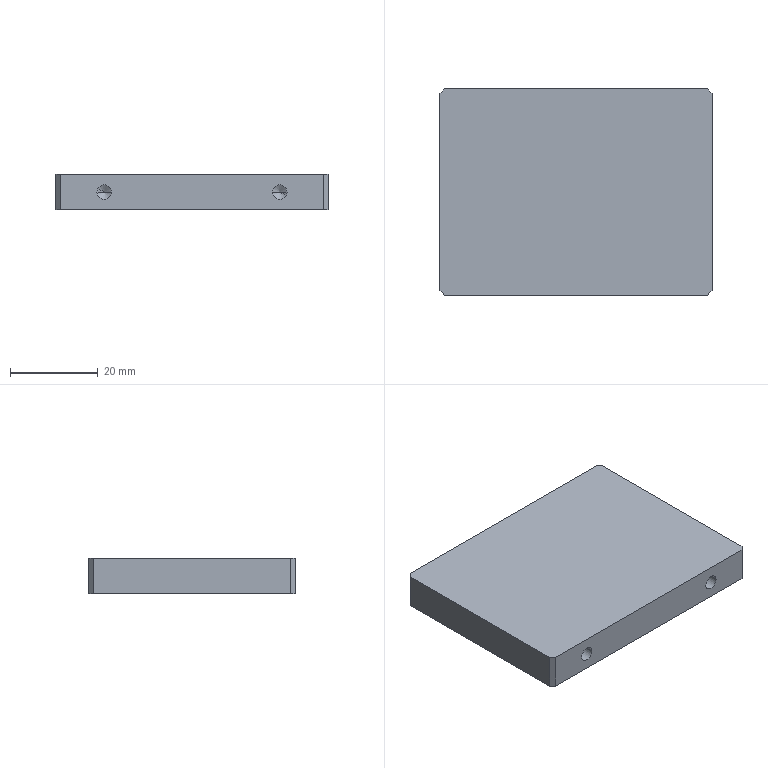CAM job | Mastercam | mm | 7 operations | part box 62 x 47 x 8
1. Facing | 24 - 100 平铣刀
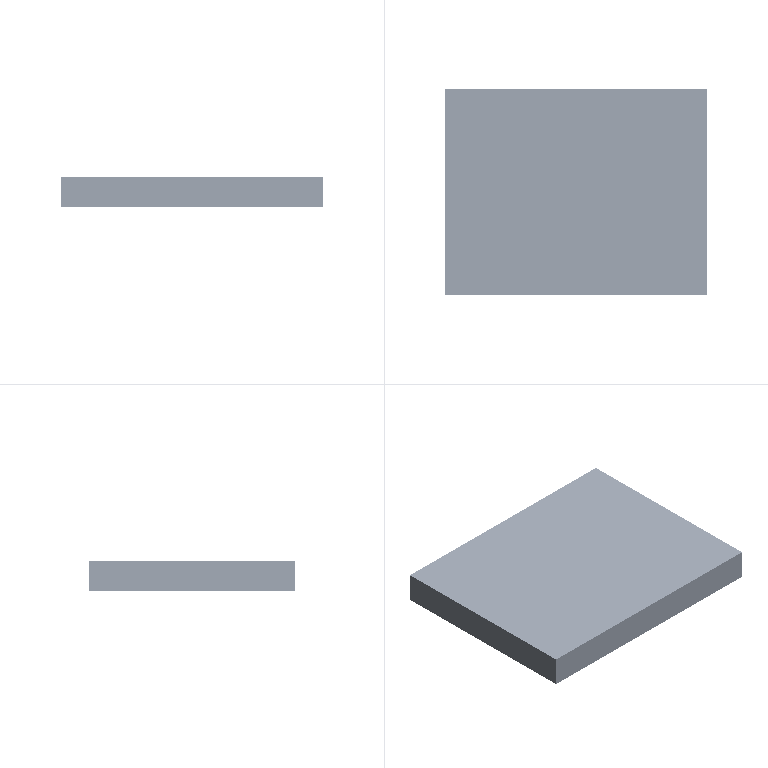2. Contour (Ramp) | 10 - 10 平铣刀
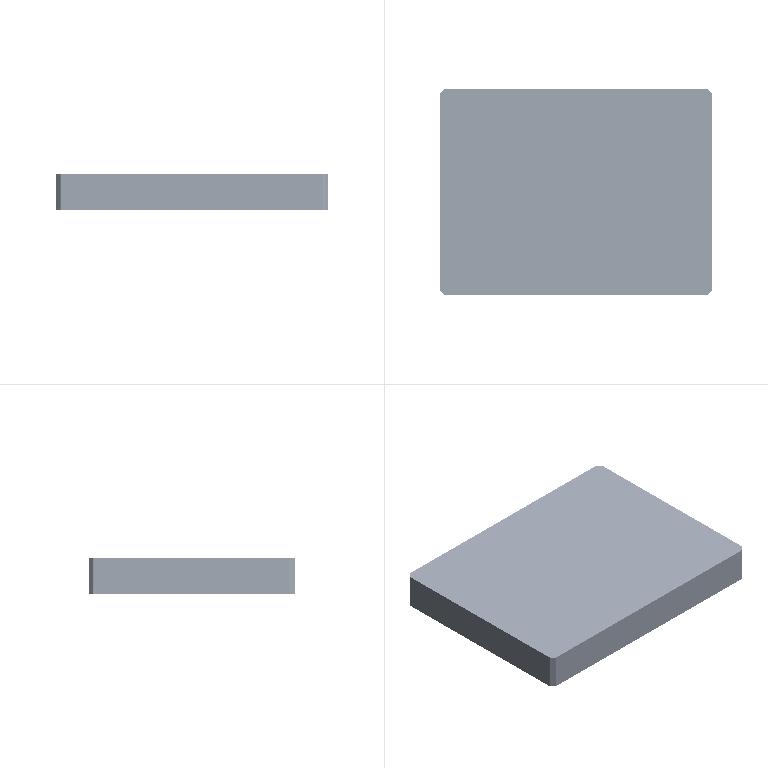3. Contour (2D) | 10 - 10 平铣刀
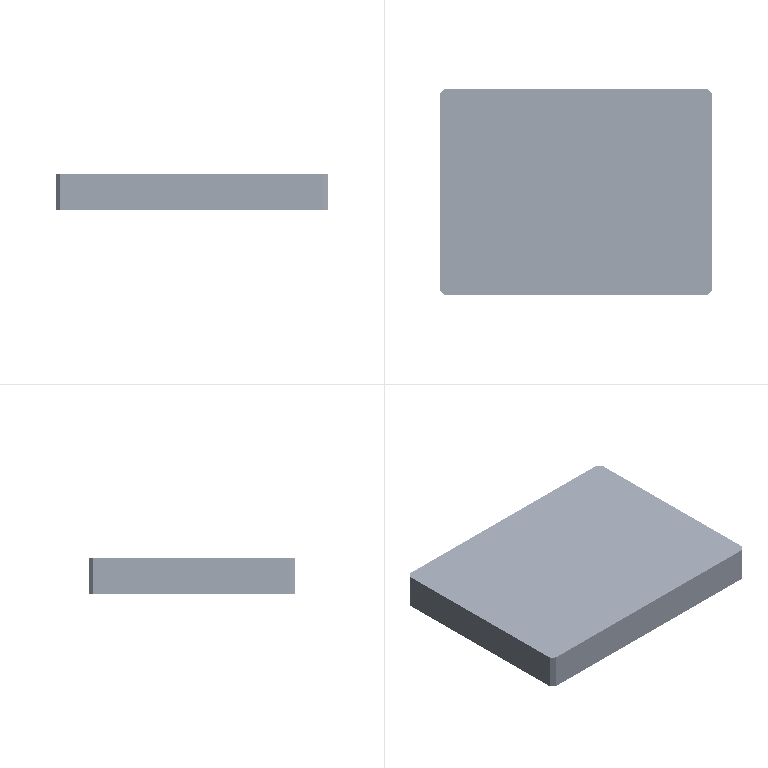4. Contour (2D chamfer) | 7 - 4 倒角刀
5. Facing | 20 - 63 平铣刀
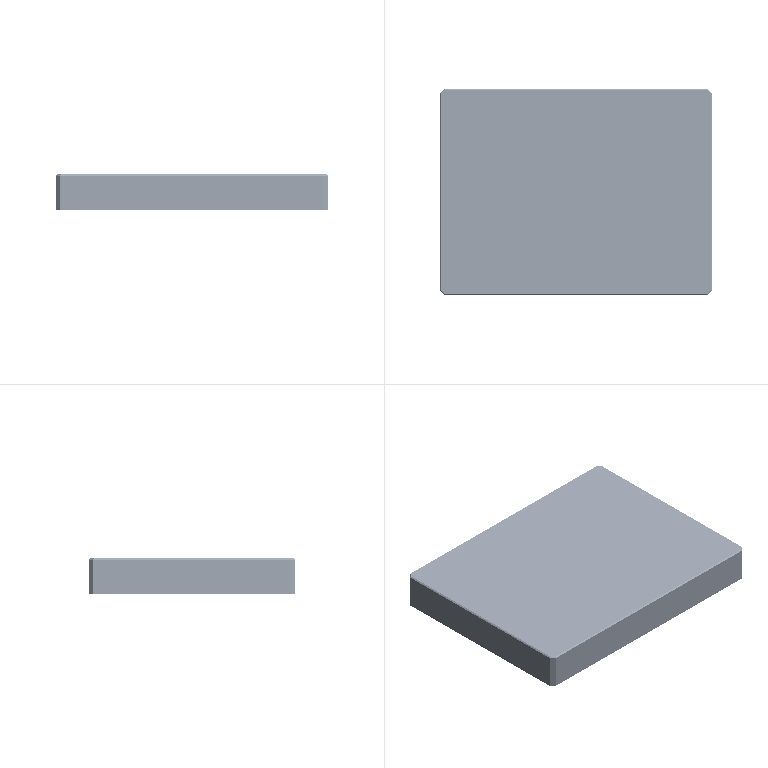6. Contour (2D chamfer) | 7 - 4 倒角刀
7. Drill/Counterbore | 7 - 4 倒角刀